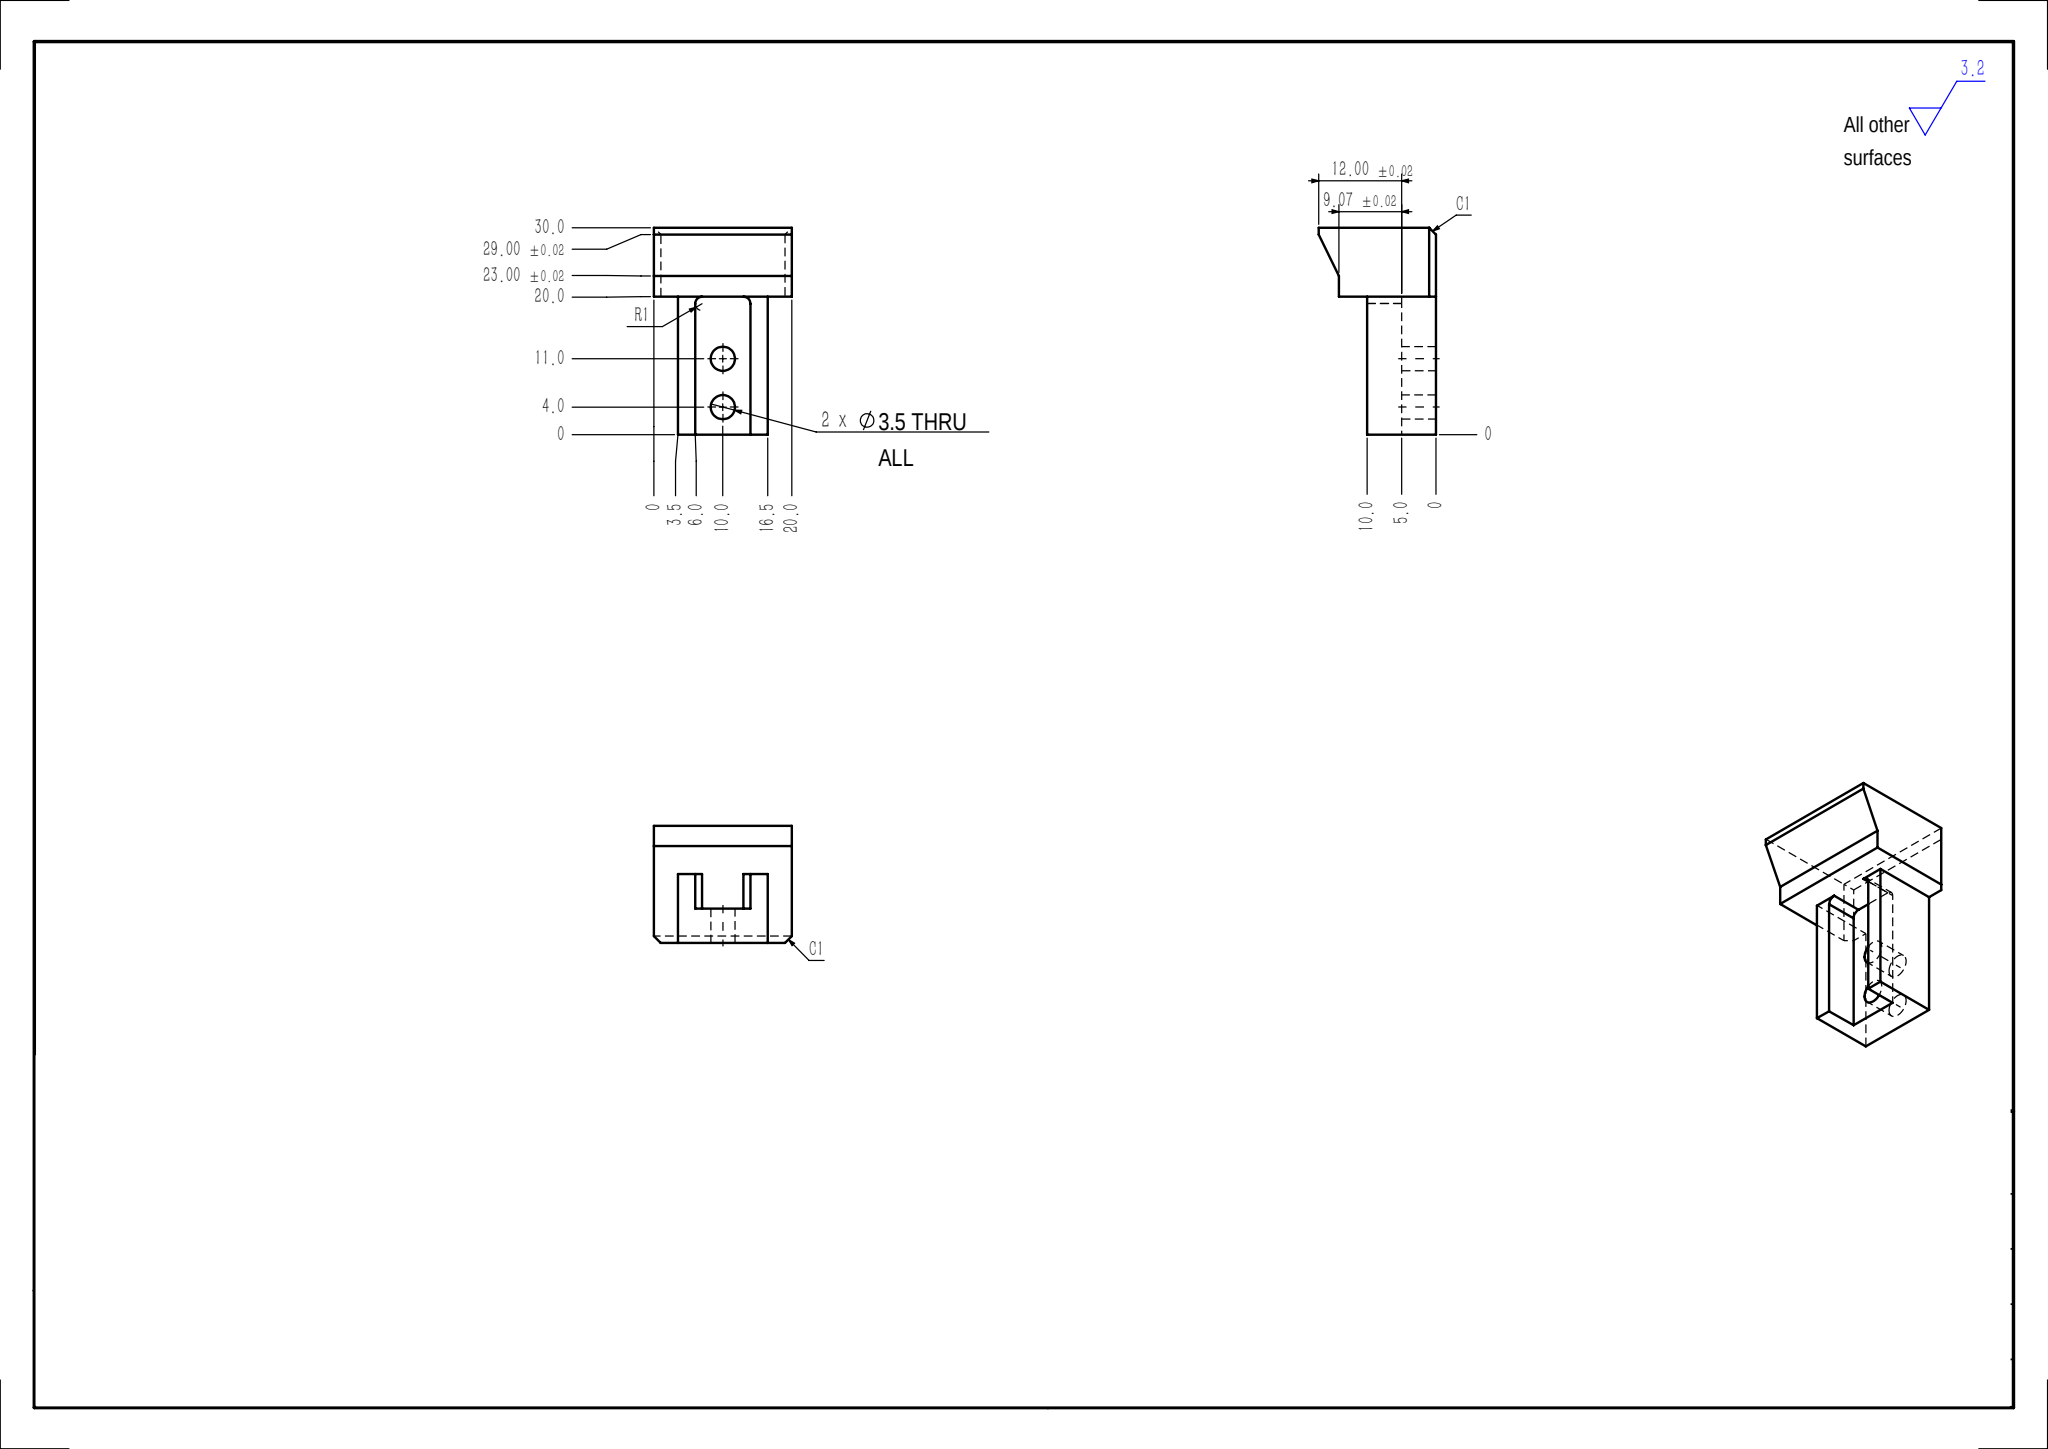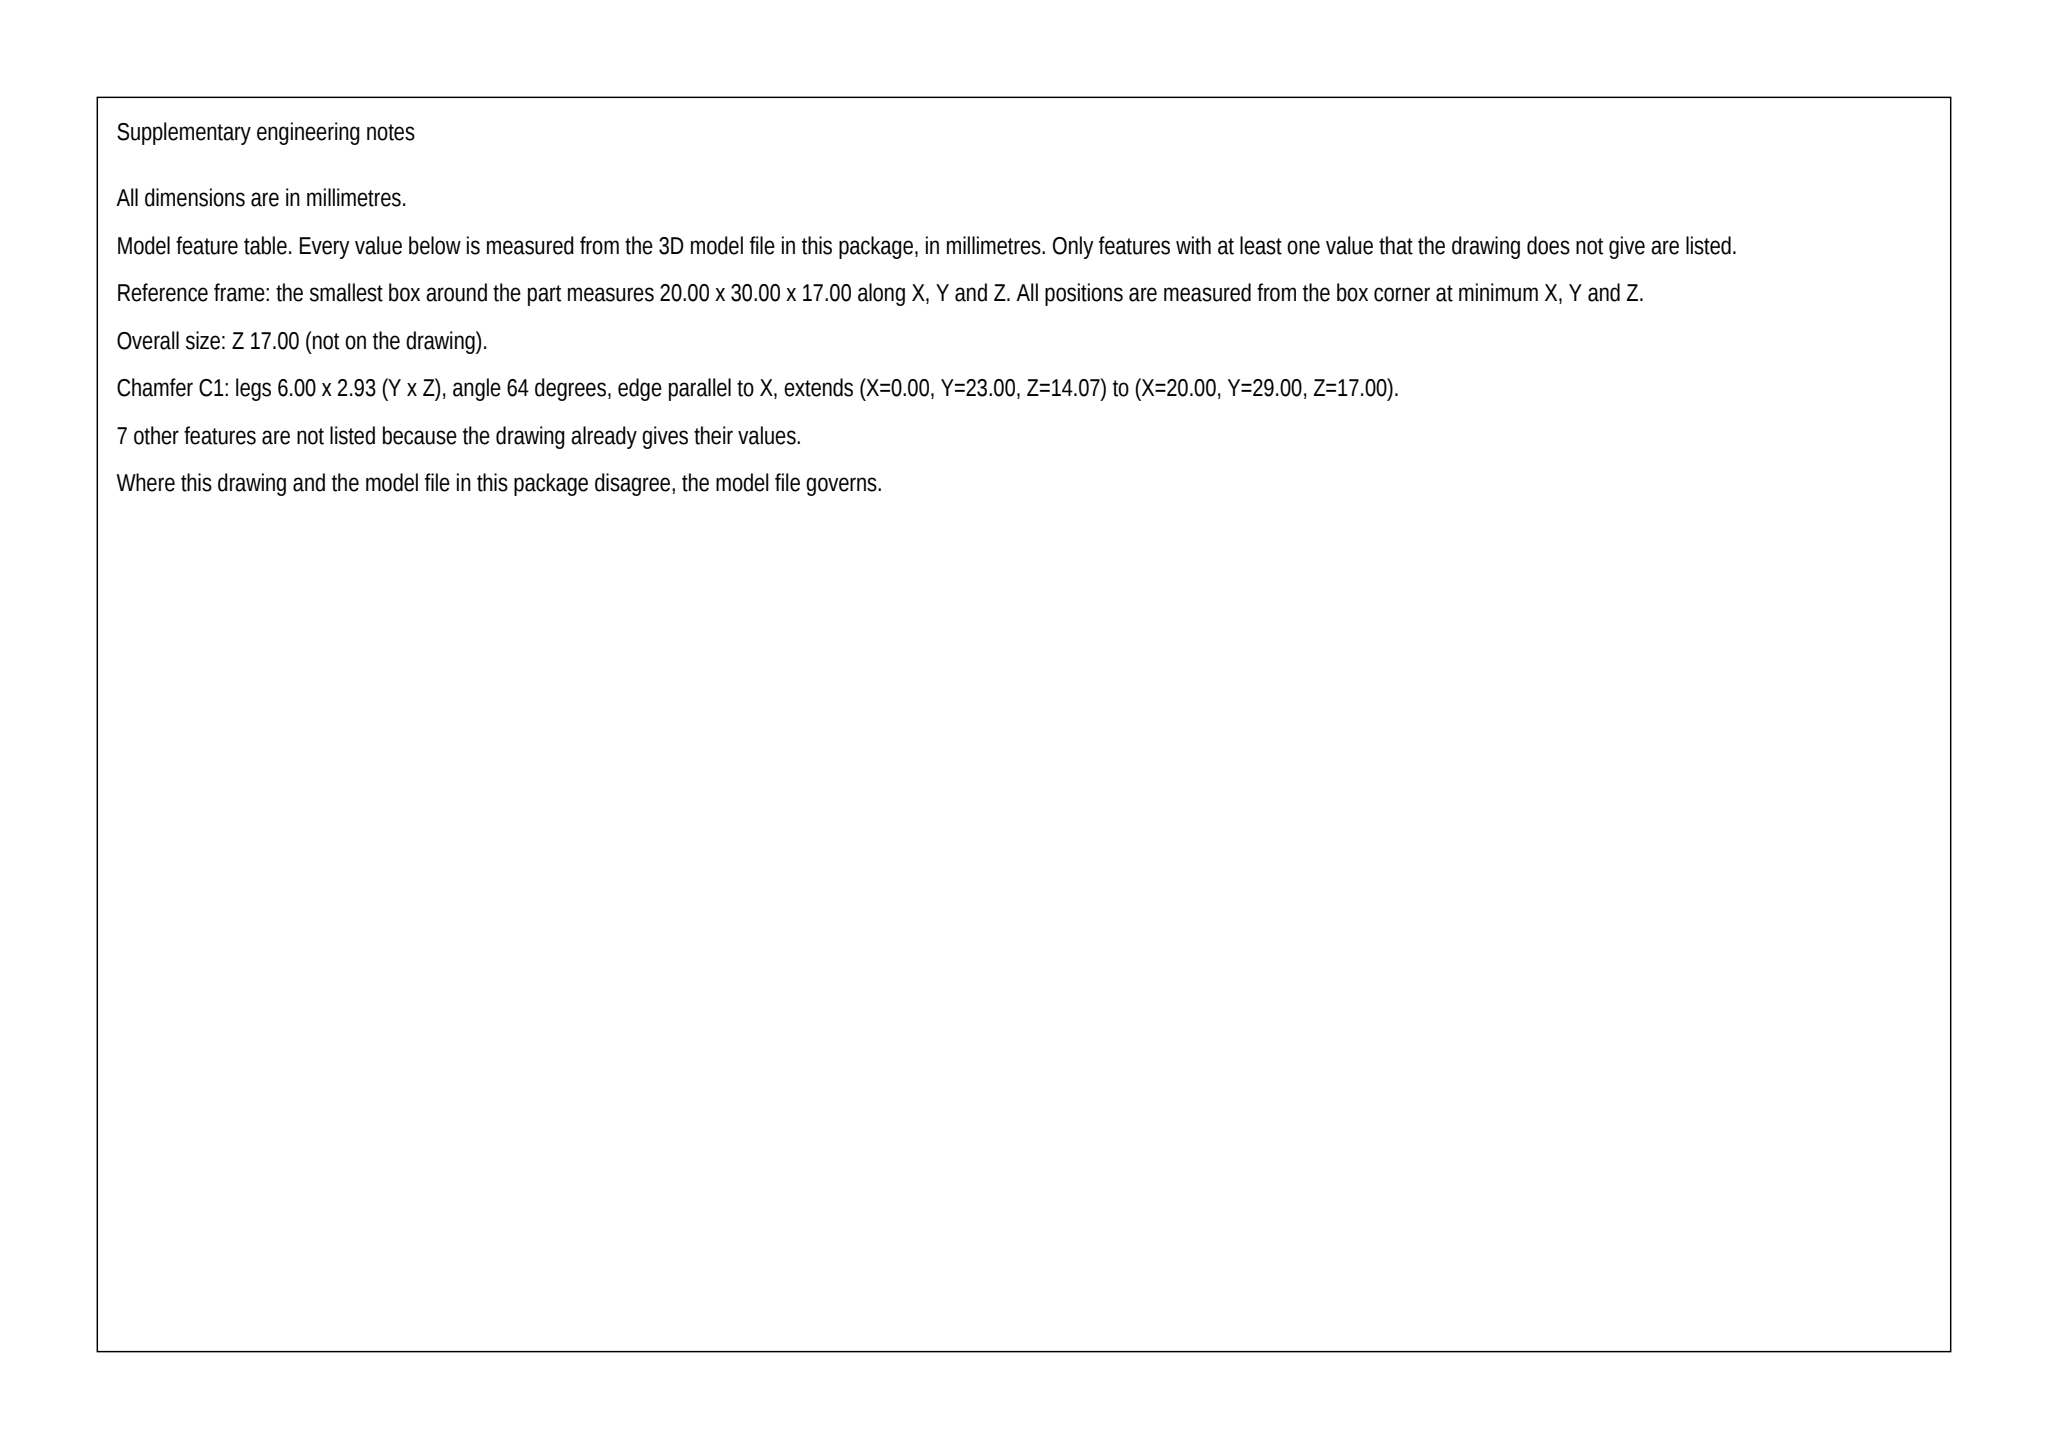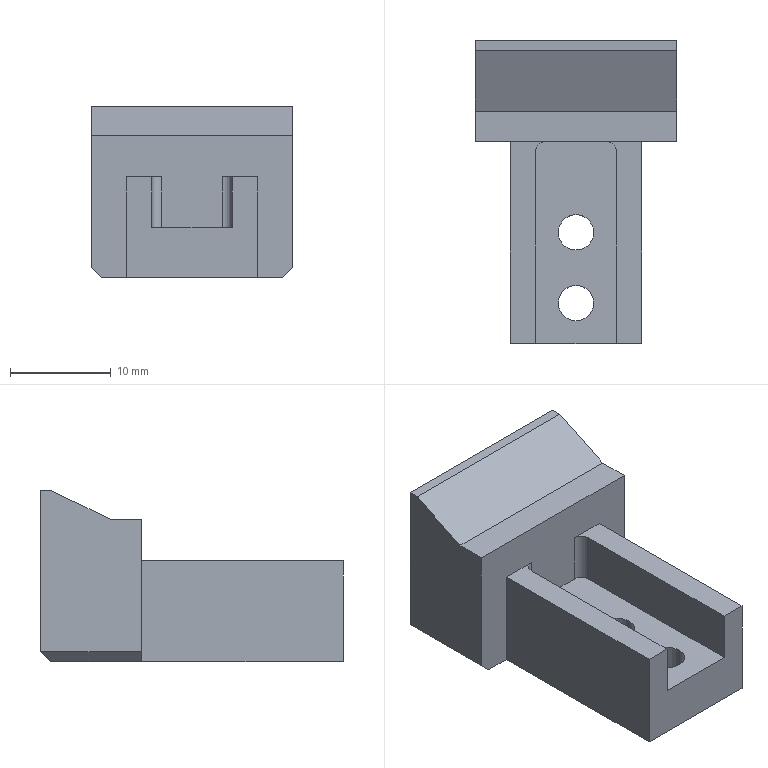Part | SolidWorks | mm | 1 solid | 25 faces | box 20 x 30 x 17 mm | volume 4735 mm3 | plane 19 | cylinder 6 | commonest cylinder face diameters 3.5 x4 2 x2
build123d program:
from build123d import *

# Parameters (mm, degrees)
SKETCH1_W                  = 20
SKETCH1_H                  = 30
BOSS_EXTRUDE1_DEPTH        = 5
SKETCH2_W                  = 8
SKETCH2_H                  = 40
CUT_EXTRUDE1_DEPTH         = 5
SKETCH3_W                  = 3.5
SKETCH3_H                  = 20
CUT_EXTRUDE2_DEPTH         = 21.616
SKETCH4_W                  = 20
SKETCH4_H                  = 10
BOSS_EXTRUDE2_DEPTH        = 8
F_3_5_3_5_DIAMETER_HOLE1_D = 3.5
CHAMFER1_SIZE              = 1
SKETCH8_W                  = 20
SKETCH8_H                  = 10
CUT_EXTRUDE4_DEPTH         = 1
FILLET3_R                  = 1
CUT_EXTRUDE5_DEPTH         = 28.731


with BuildPart() as part:
    # Sketch1 → Boss-Extrude1 (new, symmetric)
    with BuildSketch(Plane.XY):
        Rectangle(SKETCH1_W, SKETCH1_H)
    extrude(amount=BOSS_EXTRUDE1_DEPTH, both=True)

    # Sketch2 → Cut-Extrude1 (cut)
    with BuildSketch(Plane.XY.offset(5)):
        with Locations((0, -15)):
            Rectangle(SKETCH2_W, SKETCH2_H)
    extrude(amount=-CUT_EXTRUDE1_DEPTH, mode=Mode.SUBTRACT)

    # Sketch3 → Cut-Extrude2 (cut, through all)
    with BuildSketch(Plane.XY.offset(5)):
        with Locations((-8.25, -5)):
            Rectangle(SKETCH3_W, SKETCH3_H)
        with Locations((8.25, -5)):
            Rectangle(SKETCH3_W, SKETCH3_H)
    extrude(amount=-CUT_EXTRUDE2_DEPTH, mode=Mode.SUBTRACT)

    # Sketch4 → Boss-Extrude2 (add)
    with BuildSketch(Plane.XY.offset(5)):
        with Locations((0, 10)):
            Rectangle(SKETCH4_W, SKETCH4_H)
    extrude(amount=BOSS_EXTRUDE2_DEPTH)

    # 3.5 _3.5_ Diameter Hole1 (through all)
    with Locations(Plane(origin=(0, 0, -5), x_dir=(-1, 0, 0), z_dir=(0, 0, -1))):
        with Locations((0, -11), (0, -4)):
            Hole(F_3_5_3_5_DIAMETER_HOLE1_D / 2)

    # Chamfer1
    chamfer1_edges = [part.edges().sort_by_distance(p)[0] for p in [
        (10, 10, -5),
        (-10, 10, -5),
        (0, 15, -5),
    ]]
    chamfer(chamfer1_edges, length=CHAMFER1_SIZE)

    # Sketch8 → Cut-Extrude4 (cut)
    with BuildSketch(Plane.XY.offset(13)):
        with Locations((0, 10)):
            Rectangle(SKETCH8_W, SKETCH8_H)
    extrude(amount=-CUT_EXTRUDE4_DEPTH, mode=Mode.SUBTRACT)

    # Fillet3
    fillet3_edges = [part.edges().sort_by_distance(p)[0] for p in [
        (4, 5, 2.5),
        (-4, 5, 2.5),
    ]]
    fillet(fillet3_edges, radius=FILLET3_R)

    # Sketch9 → Cut-Extrude5 (cut, through all)
    with BuildSketch(Plane(origin=(10, 0, 0), x_dir=(0, 0, -1), z_dir=(1, 0, 0))):
        Polygon((-12, 14), (-9.074, 8), (-9.074, 5), (-12, 5), align=None)
    extrude(amount=-CUT_EXTRUDE5_DEPTH, mode=Mode.SUBTRACT)


solid = part.part
STEP:
#1=CARTESIAN_POINT('',(1.75,-11.,0.));
#2=VERTEX_POINT('',#1);
#3=CARTESIAN_POINT('',(-1.75,-11.,0.));
#4=VERTEX_POINT('',#3);
#5=CARTESIAN_POINT('',(-0.,-11.,0.));
#6=DIRECTION('',(0.,0.,-1.));
#7=DIRECTION('',(-1.,0.,0.));
#8=AXIS2_PLACEMENT_3D('',#5,#6,#7);
#9=CIRCLE('',#8,1.75);
#10=EDGE_CURVE('',#2,#4,#9,.T.);
#11=ORIENTED_EDGE('',*,*,#10,.F.);
#12=CARTESIAN_POINT('',(1.75,-11.,-5.));
#13=VERTEX_POINT('',#12);
#14=CARTESIAN_POINT('',(1.75,-11.,-5.));
#15=DIRECTION('',(0.,0.,-1.));
#16=VECTOR('',#15,1000.);
#17=LINE('',#14,#16);
#18=EDGE_CURVE('',#2,#13,#17,.T.);
#19=ORIENTED_EDGE('',*,*,#18,.T.);
#20=CARTESIAN_POINT('',(-1.75,-11.,-5.));
#21=VERTEX_POINT('',#20);
#22=CARTESIAN_POINT('',(-0.,-11.,-5.));
#23=DIRECTION('',(0.,0.,-1.));
#24=DIRECTION('',(-1.,0.,0.));
#25=AXIS2_PLACEMENT_3D('',#22,#23,#24);
#26=CIRCLE('',#25,1.75);
#27=EDGE_CURVE('',#13,#21,#26,.T.);
#28=ORIENTED_EDGE('',*,*,#27,.T.);
#29=CARTESIAN_POINT('',(-1.75,-11.,-5.));
#30=DIRECTION('',(0.,0.,-1.));
#31=VECTOR('',#30,1000.);
#32=LINE('',#29,#31);
#33=EDGE_CURVE('',#4,#21,#32,.T.);
#34=ORIENTED_EDGE('',*,*,#33,.F.);
#35=EDGE_LOOP('',(#11,#19,#28,#34));
#36=FACE_OUTER_BOUND('',#35,.T.);
#37=CARTESIAN_POINT('',(-0.,-11.,-5.));
#38=DIRECTION('',(0.,0.,-1.));
#39=DIRECTION('',(-1.,0.,0.));
#40=AXIS2_PLACEMENT_3D('',#37,#38,#39);
#41=CYLINDRICAL_SURFACE('',#40,1.75);
#42=ADVANCED_FACE('',(#36),#41,.F.);
#43=CARTESIAN_POINT('',(1.75,-4.,0.));
#44=VERTEX_POINT('',#43);
#45=CARTESIAN_POINT('',(-1.75,-4.,0.));
#46=VERTEX_POINT('',#45);
#47=CARTESIAN_POINT('',(0.,-4.,0.));
#48=DIRECTION('',(0.,0.,-1.));
#49=DIRECTION('',(-1.,0.,0.));
#50=AXIS2_PLACEMENT_3D('',#47,#48,#49);
#51=CIRCLE('',#50,1.75);
#52=EDGE_CURVE('',#44,#46,#51,.T.);
#53=ORIENTED_EDGE('',*,*,#52,.F.);
#54=CARTESIAN_POINT('',(1.75,-4.,-5.));
#55=VERTEX_POINT('',#54);
#56=CARTESIAN_POINT('',(1.75,-4.,-5.));
#57=DIRECTION('',(0.,0.,-1.));
#58=VECTOR('',#57,1000.);
#59=LINE('',#56,#58);
#60=EDGE_CURVE('',#44,#55,#59,.T.);
#61=ORIENTED_EDGE('',*,*,#60,.T.);
#62=CARTESIAN_POINT('',(-1.75,-4.,-5.));
#63=VERTEX_POINT('',#62);
#64=CARTESIAN_POINT('',(0.,-4.,-5.));
#65=DIRECTION('',(0.,0.,-1.));
#66=DIRECTION('',(-1.,0.,0.));
#67=AXIS2_PLACEMENT_3D('',#64,#65,#66);
#68=CIRCLE('',#67,1.75);
#69=EDGE_CURVE('',#55,#63,#68,.T.);
#70=ORIENTED_EDGE('',*,*,#69,.T.);
#71=CARTESIAN_POINT('',(-1.75,-4.,-5.));
#72=DIRECTION('',(0.,0.,-1.));
#73=VECTOR('',#72,1000.);
#74=LINE('',#71,#73);
#75=EDGE_CURVE('',#46,#63,#74,.T.);
#76=ORIENTED_EDGE('',*,*,#75,.F.);
#77=EDGE_LOOP('',(#53,#61,#70,#76));
#78=FACE_OUTER_BOUND('',#77,.T.);
#79=CARTESIAN_POINT('',(0.,-4.,-5.));
#80=DIRECTION('',(0.,0.,-1.));
#81=DIRECTION('',(-1.,0.,0.));
#82=AXIS2_PLACEMENT_3D('',#79,#80,#81);
#83=CYLINDRICAL_SURFACE('',#82,1.75);
#84=ADVANCED_FACE('',(#78),#83,.F.);
#85=CARTESIAN_POINT('',(10.,14.,12.));
#86=VERTEX_POINT('',#85);
#87=CARTESIAN_POINT('',(10.,15.,12.));
#88=VERTEX_POINT('',#87);
#89=CARTESIAN_POINT('',(10.,15.,12.));
#90=DIRECTION('',(0.,1.,0.));
#91=VECTOR('',#90,1000.);
#92=LINE('',#89,#91);
#93=EDGE_CURVE('',#86,#88,#92,.T.);
#94=ORIENTED_EDGE('',*,*,#93,.F.);
#95=CARTESIAN_POINT('',(10.,8.,9.074));
#96=VERTEX_POINT('',#95);
#97=CARTESIAN_POINT('',(10.,14.,12.));
#98=DIRECTION('',(0.,0.8988,0.4384));
#99=VECTOR('',#98,1000.);
#100=LINE('',#97,#99);
#101=EDGE_CURVE('',#96,#86,#100,.T.);
#102=ORIENTED_EDGE('',*,*,#101,.F.);
#103=CARTESIAN_POINT('',(10.,5.,9.074));
#104=VERTEX_POINT('',#103);
#105=CARTESIAN_POINT('',(10.,8.,9.074));
#106=DIRECTION('',(-0.,1.,0.));
#107=VECTOR('',#106,1000.);
#108=LINE('',#105,#107);
#109=EDGE_CURVE('',#104,#96,#108,.T.);
#110=ORIENTED_EDGE('',*,*,#109,.F.);
#111=CARTESIAN_POINT('',(10.,5.,-4.));
#112=VERTEX_POINT('',#111);
#113=CARTESIAN_POINT('',(10.,5.,-5.));
#114=DIRECTION('',(0.,0.,1.));
#115=VECTOR('',#114,1000.);
#116=LINE('',#113,#115);
#117=EDGE_CURVE('',#112,#104,#116,.T.);
#118=ORIENTED_EDGE('',*,*,#117,.F.);
#119=CARTESIAN_POINT('',(10.,15.,-4.));
#120=VERTEX_POINT('',#119);
#121=CARTESIAN_POINT('',(10.,15.,-4.));
#122=DIRECTION('',(-0.,1.,0.));
#123=VECTOR('',#122,1000.);
#124=LINE('',#121,#123);
#125=EDGE_CURVE('',#112,#120,#124,.T.);
#126=ORIENTED_EDGE('',*,*,#125,.T.);
#127=CARTESIAN_POINT('',(10.,15.,5.));
#128=DIRECTION('',(0.,0.,-1.));
#129=VECTOR('',#128,1000.);
#130=LINE('',#127,#129);
#131=EDGE_CURVE('',#88,#120,#130,.T.);
#132=ORIENTED_EDGE('',*,*,#131,.F.);
#133=EDGE_LOOP('',(#94,#102,#110,#118,#126,#132));
#134=FACE_OUTER_BOUND('',#133,.T.);
#135=CARTESIAN_POINT('',(10.,15.,5.));
#136=DIRECTION('',(-1.,-0.,0.));
#137=DIRECTION('',(0.,-1.,0.));
#138=AXIS2_PLACEMENT_3D('',#135,#136,#137);
#139=PLANE('',#138);
#140=ADVANCED_FACE('',(#134),#139,.F.);
#141=CARTESIAN_POINT('',(-10.,15.,12.));
#142=VERTEX_POINT('',#141);
#143=CARTESIAN_POINT('',(-10.,15.,12.));
#144=DIRECTION('',(-1.,0.,0.));
#145=VECTOR('',#144,1000.);
#146=LINE('',#143,#145);
#147=EDGE_CURVE('',#88,#142,#146,.T.);
#148=ORIENTED_EDGE('',*,*,#147,.F.);
#149=ORIENTED_EDGE('',*,*,#131,.T.);
#150=CARTESIAN_POINT('',(-10.,15.,-4.));
#151=VERTEX_POINT('',#150);
#152=CARTESIAN_POINT('',(-10.,15.,-4.));
#153=DIRECTION('',(-1.,0.,0.));
#154=VECTOR('',#153,1000.);
#155=LINE('',#152,#154);
#156=EDGE_CURVE('',#120,#151,#155,.T.);
#157=ORIENTED_EDGE('',*,*,#156,.T.);
#158=CARTESIAN_POINT('',(-10.,15.,5.));
#159=DIRECTION('',(0.,0.,-1.));
#160=VECTOR('',#159,1000.);
#161=LINE('',#158,#160);
#162=EDGE_CURVE('',#142,#151,#161,.T.);
#163=ORIENTED_EDGE('',*,*,#162,.F.);
#164=EDGE_LOOP('',(#148,#149,#157,#163));
#165=FACE_OUTER_BOUND('',#164,.T.);
#166=CARTESIAN_POINT('',(-10.,15.,5.));
#167=DIRECTION('',(0.,-1.,0.));
#168=DIRECTION('',(0.,0.,-1.));
#169=AXIS2_PLACEMENT_3D('',#166,#167,#168);
#170=PLANE('',#169);
#171=ADVANCED_FACE('',(#165),#170,.F.);
#172=CARTESIAN_POINT('',(-10.,5.,9.074));
#173=VERTEX_POINT('',#172);
#174=CARTESIAN_POINT('',(-10.,8.,9.074));
#175=VERTEX_POINT('',#174);
#176=CARTESIAN_POINT('',(-10.,8.,9.074));
#177=DIRECTION('',(-0.,1.,0.));
#178=VECTOR('',#177,1000.);
#179=LINE('',#176,#178);
#180=EDGE_CURVE('',#173,#175,#179,.T.);
#181=ORIENTED_EDGE('',*,*,#180,.T.);
#182=CARTESIAN_POINT('',(-10.,14.,12.));
#183=VERTEX_POINT('',#182);
#184=CARTESIAN_POINT('',(-10.,14.,12.));
#185=DIRECTION('',(0.,0.8988,0.4384));
#186=VECTOR('',#185,1000.);
#187=LINE('',#184,#186);
#188=EDGE_CURVE('',#175,#183,#187,.T.);
#189=ORIENTED_EDGE('',*,*,#188,.T.);
#190=CARTESIAN_POINT('',(-10.,15.,12.));
#191=DIRECTION('',(0.,-1.,0.));
#192=VECTOR('',#191,1000.);
#193=LINE('',#190,#192);
#194=EDGE_CURVE('',#142,#183,#193,.T.);
#195=ORIENTED_EDGE('',*,*,#194,.F.);
#196=ORIENTED_EDGE('',*,*,#162,.T.);
#197=CARTESIAN_POINT('',(-10.,5.,-4.));
#198=VERTEX_POINT('',#197);
#199=CARTESIAN_POINT('',(-10.,15.,-4.));
#200=DIRECTION('',(0.,-1.,0.));
#201=VECTOR('',#200,1000.);
#202=LINE('',#199,#201);
#203=EDGE_CURVE('',#151,#198,#202,.T.);
#204=ORIENTED_EDGE('',*,*,#203,.T.);
#205=CARTESIAN_POINT('',(-10.,5.,-5.));
#206=DIRECTION('',(0.,0.,1.));
#207=VECTOR('',#206,1000.);
#208=LINE('',#205,#207);
#209=EDGE_CURVE('',#198,#173,#208,.T.);
#210=ORIENTED_EDGE('',*,*,#209,.T.);
#211=EDGE_LOOP('',(#181,#189,#195,#196,#204,#210));
#212=FACE_OUTER_BOUND('',#211,.T.);
#213=CARTESIAN_POINT('',(-10.,15.,5.));
#214=DIRECTION('',(1.,0.,0.));
#215=DIRECTION('',(-0.,1.,0.));
#216=AXIS2_PLACEMENT_3D('',#213,#214,#215);
#217=PLANE('',#216);
#218=ADVANCED_FACE('',(#212),#217,.F.);
#219=ORIENTED_EDGE('',*,*,#117,.T.);
#220=CARTESIAN_POINT('',(-10.,5.,9.074));
#221=DIRECTION('',(1.,0.,0.));
#222=VECTOR('',#221,1000.);
#223=LINE('',#220,#222);
#224=EDGE_CURVE('',#173,#104,#223,.T.);
#225=ORIENTED_EDGE('',*,*,#224,.F.);
#226=ORIENTED_EDGE('',*,*,#209,.F.);
#227=CARTESIAN_POINT('',(-9.,5.,-5.));
#228=VERTEX_POINT('',#227);
#229=CARTESIAN_POINT('',(-10.,5.,-4.));
#230=DIRECTION('',(0.7071,0.,-0.7071));
#231=VECTOR('',#230,1000.);
#232=LINE('',#229,#231);
#233=EDGE_CURVE('',#198,#228,#232,.T.);
#234=ORIENTED_EDGE('',*,*,#233,.T.);
#235=CARTESIAN_POINT('',(-6.5,5.,-5.));
#236=VERTEX_POINT('',#235);
#237=CARTESIAN_POINT('',(-10.,5.,-5.));
#238=DIRECTION('',(-1.,0.,0.));
#239=VECTOR('',#238,1000.);
#240=LINE('',#237,#239);
#241=EDGE_CURVE('',#236,#228,#240,.T.);
#242=ORIENTED_EDGE('',*,*,#241,.F.);
#243=CARTESIAN_POINT('',(-6.5,5.,5.));
#244=VERTEX_POINT('',#243);
#245=CARTESIAN_POINT('',(-6.5,5.,-5.));
#246=DIRECTION('',(0.,0.,1.));
#247=VECTOR('',#246,1000.);
#248=LINE('',#245,#247);
#249=EDGE_CURVE('',#236,#244,#248,.T.);
#250=ORIENTED_EDGE('',*,*,#249,.T.);
#251=CARTESIAN_POINT('',(-3.,5.,5.));
#252=VERTEX_POINT('',#251);
#253=CARTESIAN_POINT('',(-10.,5.,5.));
#254=DIRECTION('',(1.,0.,0.));
#255=VECTOR('',#254,1000.);
#256=LINE('',#253,#255);
#257=EDGE_CURVE('',#244,#252,#256,.T.);
#258=ORIENTED_EDGE('',*,*,#257,.T.);
#259=CARTESIAN_POINT('',(-3.,5.,0.));
#260=VERTEX_POINT('',#259);
#261=CARTESIAN_POINT('',(-3.,5.,0.));
#262=DIRECTION('',(0.,0.,-1.));
#263=VECTOR('',#262,1000.);
#264=LINE('',#261,#263);
#265=EDGE_CURVE('',#252,#260,#264,.T.);
#266=ORIENTED_EDGE('',*,*,#265,.T.);
#267=CARTESIAN_POINT('',(3.,5.,0.));
#268=VERTEX_POINT('',#267);
#269=CARTESIAN_POINT('',(-4.,5.,0.));
#270=DIRECTION('',(-1.,-0.,0.));
#271=VECTOR('',#270,1000.);
#272=LINE('',#269,#271);
#273=EDGE_CURVE('',#268,#260,#272,.T.);
#274=ORIENTED_EDGE('',*,*,#273,.F.);
#275=CARTESIAN_POINT('',(3.,5.,5.));
#276=VERTEX_POINT('',#275);
#277=CARTESIAN_POINT('',(3.,5.,5.));
#278=DIRECTION('',(0.,0.,1.));
#279=VECTOR('',#278,1000.);
#280=LINE('',#277,#279);
#281=EDGE_CURVE('',#268,#276,#280,.T.);
#282=ORIENTED_EDGE('',*,*,#281,.T.);
#283=CARTESIAN_POINT('',(6.5,5.,5.));
#284=VERTEX_POINT('',#283);
#285=CARTESIAN_POINT('',(-10.,5.,5.));
#286=DIRECTION('',(1.,0.,0.));
#287=VECTOR('',#286,1000.);
#288=LINE('',#285,#287);
#289=EDGE_CURVE('',#276,#284,#288,.T.);
#290=ORIENTED_EDGE('',*,*,#289,.T.);
#291=CARTESIAN_POINT('',(6.5,5.,-5.));
#292=VERTEX_POINT('',#291);
#293=CARTESIAN_POINT('',(6.5,5.,-5.));
#294=DIRECTION('',(0.,0.,1.));
#295=VECTOR('',#294,1000.);
#296=LINE('',#293,#295);
#297=EDGE_CURVE('',#292,#284,#296,.T.);
#298=ORIENTED_EDGE('',*,*,#297,.F.);
#299=CARTESIAN_POINT('',(9.,5.,-5.));
#300=VERTEX_POINT('',#299);
#301=CARTESIAN_POINT('',(10.,5.,-5.));
#302=DIRECTION('',(-1.,0.,0.));
#303=VECTOR('',#302,1000.);
#304=LINE('',#301,#303);
#305=EDGE_CURVE('',#300,#292,#304,.T.);
#306=ORIENTED_EDGE('',*,*,#305,.F.);
#307=CARTESIAN_POINT('',(10.,5.,-4.));
#308=DIRECTION('',(0.7071,0.,0.7071));
#309=VECTOR('',#308,1000.);
#310=LINE('',#307,#309);
#311=EDGE_CURVE('',#300,#112,#310,.T.);
#312=ORIENTED_EDGE('',*,*,#311,.T.);
#313=EDGE_LOOP('',(#219,#225,#226,#234,#242,#250,#258,#266,#274,#282,#290,#298,#306,#312));
#314=FACE_OUTER_BOUND('',#313,.T.);
#315=CARTESIAN_POINT('',(-4.,5.,0.));
#316=DIRECTION('',(-0.,1.,0.));
#317=DIRECTION('',(-1.,-0.,0.));
#318=AXIS2_PLACEMENT_3D('',#315,#316,#317);
#319=PLANE('',#318);
#320=ADVANCED_FACE('',(#314),#319,.F.);
#321=ORIENTED_EDGE('',*,*,#257,.F.);
#322=CARTESIAN_POINT('',(-6.5,-15.,5.));
#323=VERTEX_POINT('',#322);
#324=CARTESIAN_POINT('',(-6.5,-15.,5.));
#325=DIRECTION('',(0.,1.,0.));
#326=VECTOR('',#325,1000.);
#327=LINE('',#324,#326);
#328=EDGE_CURVE('',#323,#244,#327,.T.);
#329=ORIENTED_EDGE('',*,*,#328,.F.);
#330=CARTESIAN_POINT('',(-4.,-15.,5.));
#331=VERTEX_POINT('',#330);
#332=CARTESIAN_POINT('',(-10.,-15.,5.));
#333=DIRECTION('',(1.,0.,0.));
#334=VECTOR('',#333,1000.);
#335=LINE('',#332,#334);
#336=EDGE_CURVE('',#323,#331,#335,.T.);
#337=ORIENTED_EDGE('',*,*,#336,.T.);
#338=CARTESIAN_POINT('',(-4.,4.,5.));
#339=VERTEX_POINT('',#338);
#340=CARTESIAN_POINT('',(-4.,-35.,5.));
#341=DIRECTION('',(0.,-1.,0.));
#342=VECTOR('',#341,1000.);
#343=LINE('',#340,#342);
#344=EDGE_CURVE('',#339,#331,#343,.T.);
#345=ORIENTED_EDGE('',*,*,#344,.F.);
#346=CARTESIAN_POINT('',(-3.,4.,5.));
#347=DIRECTION('',(0.,0.,-1.));
#348=DIRECTION('',(1.,0.,0.));
#349=AXIS2_PLACEMENT_3D('',#346,#347,#348);
#350=CIRCLE('',#349,1.);
#351=EDGE_CURVE('',#339,#252,#350,.T.);
#352=ORIENTED_EDGE('',*,*,#351,.T.);
#353=EDGE_LOOP('',(#321,#329,#337,#345,#352));
#354=FACE_OUTER_BOUND('',#353,.T.);
#355=CARTESIAN_POINT('',(0.,0.,5.));
#356=DIRECTION('',(0.,0.,1.));
#357=DIRECTION('',(1.,0.,0.));
#358=AXIS2_PLACEMENT_3D('',#355,#356,#357);
#359=PLANE('',#358);
#360=ADVANCED_FACE('',(#354),#359,.T.);
#361=ORIENTED_EDGE('',*,*,#336,.F.);
#362=CARTESIAN_POINT('',(-6.5,-15.,-5.));
#363=VERTEX_POINT('',#362);
#364=CARTESIAN_POINT('',(-6.5,-15.,-5.));
#365=DIRECTION('',(0.,0.,1.));
#366=VECTOR('',#365,1000.);
#367=LINE('',#364,#366);
#368=EDGE_CURVE('',#363,#323,#367,.T.);
#369=ORIENTED_EDGE('',*,*,#368,.F.);
#370=CARTESIAN_POINT('',(6.5,-15.,-5.));
#371=VERTEX_POINT('',#370);
#372=CARTESIAN_POINT('',(-10.,-15.,-5.));
#373=DIRECTION('',(1.,0.,0.));
#374=VECTOR('',#373,1000.);
#375=LINE('',#372,#374);
#376=EDGE_CURVE('',#363,#371,#375,.T.);
#377=ORIENTED_EDGE('',*,*,#376,.T.);
#378=CARTESIAN_POINT('',(6.5,-15.,5.));
#379=VERTEX_POINT('',#378);
#380=CARTESIAN_POINT('',(6.5,-15.,-5.));
#381=DIRECTION('',(0.,0.,1.));
#382=VECTOR('',#381,1000.);
#383=LINE('',#380,#382);
#384=EDGE_CURVE('',#371,#379,#383,.T.);
#385=ORIENTED_EDGE('',*,*,#384,.T.);
#386=CARTESIAN_POINT('',(4.,-15.,5.));
#387=VERTEX_POINT('',#386);
#388=CARTESIAN_POINT('',(-10.,-15.,5.));
#389=DIRECTION('',(1.,0.,0.));
#390=VECTOR('',#389,1000.);
#391=LINE('',#388,#390);
#392=EDGE_CURVE('',#387,#379,#391,.T.);
#393=ORIENTED_EDGE('',*,*,#392,.F.);
#394=CARTESIAN_POINT('',(4.,-15.,0.));
#395=VERTEX_POINT('',#394);
#396=CARTESIAN_POINT('',(4.,-15.,5.));
#397=DIRECTION('',(0.,0.,-1.));
#398=VECTOR('',#397,1000.);
#399=LINE('',#396,#398);
#400=EDGE_CURVE('',#387,#395,#399,.T.);
#401=ORIENTED_EDGE('',*,*,#400,.T.);
#402=CARTESIAN_POINT('',(-4.,-15.,0.));
#403=VERTEX_POINT('',#402);
#404=CARTESIAN_POINT('',(-10.,-15.,0.));
#405=DIRECTION('',(-1.,0.,0.));
#406=VECTOR('',#405,1000.);
#407=LINE('',#404,#406);
#408=EDGE_CURVE('',#395,#403,#407,.T.);
#409=ORIENTED_EDGE('',*,*,#408,.T.);
#410=CARTESIAN_POINT('',(-4.,-15.,5.));
#411=DIRECTION('',(0.,0.,1.));
#412=VECTOR('',#411,1000.);
#413=LINE('',#410,#412);
#414=EDGE_CURVE('',#403,#331,#413,.T.);
#415=ORIENTED_EDGE('',*,*,#414,.T.);
#416=EDGE_LOOP('',(#361,#369,#377,#385,#393,#401,#409,#415));
#417=FACE_OUTER_BOUND('',#416,.T.);
#418=CARTESIAN_POINT('',(-10.,-15.,5.));
#419=DIRECTION('',(0.,1.,0.));
#420=DIRECTION('',(0.,0.,1.));
#421=AXIS2_PLACEMENT_3D('',#418,#419,#420);
#422=PLANE('',#421);
#423=ADVANCED_FACE('',(#417),#422,.F.);
#424=ORIENTED_EDGE('',*,*,#289,.F.);
#425=CARTESIAN_POINT('',(4.,4.,5.));
#426=VERTEX_POINT('',#425);
#427=CARTESIAN_POINT('',(3.,4.,5.));
#428=DIRECTION('',(0.,0.,-1.));
#429=DIRECTION('',(1.,0.,0.));
#430=AXIS2_PLACEMENT_3D('',#427,#428,#429);
#431=CIRCLE('',#430,1.);
#432=EDGE_CURVE('',#276,#426,#431,.T.);
#433=ORIENTED_EDGE('',*,*,#432,.T.);
#434=CARTESIAN_POINT('',(4.,0.,5.));
#435=DIRECTION('',(0.,1.,0.));
#436=VECTOR('',#435,1000.);
#437=LINE('',#434,#436);
#438=EDGE_CURVE('',#387,#426,#437,.T.);
#439=ORIENTED_EDGE('',*,*,#438,.F.);
#440=ORIENTED_EDGE('',*,*,#392,.T.);
#441=CARTESIAN_POINT('',(6.5,-15.,5.));
#442=DIRECTION('',(0.,-1.,0.));
#443=VECTOR('',#442,1000.);
#444=LINE('',#441,#443);
#445=EDGE_CURVE('',#284,#379,#444,.T.);
#446=ORIENTED_EDGE('',*,*,#445,.F.);
#447=EDGE_LOOP('',(#424,#433,#439,#440,#446));
#448=FACE_OUTER_BOUND('',#447,.T.);
#449=CARTESIAN_POINT('',(0.,0.,5.));
#450=DIRECTION('',(0.,0.,1.));
#451=DIRECTION('',(1.,0.,0.));
#452=AXIS2_PLACEMENT_3D('',#449,#450,#451);
#453=PLANE('',#452);
#454=ADVANCED_FACE('',(#448),#453,.T.);
#455=CARTESIAN_POINT('',(-0.,-11.,-5.));
#456=DIRECTION('',(0.,0.,-1.));
#457=DIRECTION('',(-1.,0.,0.));
#458=AXIS2_PLACEMENT_3D('',#455,#456,#457);
#459=CIRCLE('',#458,1.75);
#460=EDGE_CURVE('',#21,#13,#459,.T.);
#461=ORIENTED_EDGE('',*,*,#460,.F.);
#462=ORIENTED_EDGE('',*,*,#27,.F.);
#463=EDGE_LOOP('',(#461,#462));
#464=FACE_BOUND('',#463,.T.);
#465=CARTESIAN_POINT('',(0.,-4.,-5.));
#466=DIRECTION('',(0.,0.,-1.));
#467=DIRECTION('',(-1.,0.,0.));
#468=AXIS2_PLACEMENT_3D('',#465,#466,#467);
#469=CIRCLE('',#468,1.75);
#470=EDGE_CURVE('',#63,#55,#469,.T.);
#471=ORIENTED_EDGE('',*,*,#470,.F.);
#472=ORIENTED_EDGE('',*,*,#69,.F.);
#473=EDGE_LOOP('',(#471,#472));
#474=FACE_BOUND('',#473,.T.);
#475=CARTESIAN_POINT('',(-9.,14.,-5.));
#476=VERTEX_POINT('',#475);
#477=CARTESIAN_POINT('',(9.,14.,-5.));
#478=VERTEX_POINT('',#477);
#479=CARTESIAN_POINT('',(0.,14.,-5.));
#480=DIRECTION('',(1.,0.,0.));
#481=VECTOR('',#480,1000.);
#482=LINE('',#479,#481);
#483=EDGE_CURVE('',#476,#478,#482,.T.);
#484=ORIENTED_EDGE('',*,*,#483,.T.);
#485=CARTESIAN_POINT('',(9.,0.,-5.));
#486=DIRECTION('',(0.,-1.,0.));
#487=VECTOR('',#486,1000.);
#488=LINE('',#485,#487);
#489=EDGE_CURVE('',#478,#300,#488,.T.);
#490=ORIENTED_EDGE('',*,*,#489,.T.);
#491=ORIENTED_EDGE('',*,*,#305,.T.);
#492=CARTESIAN_POINT('',(6.5,-15.,-5.));
#493=DIRECTION('',(0.,-1.,0.));
#494=VECTOR('',#493,1000.);
#495=LINE('',#492,#494);
#496=EDGE_CURVE('',#292,#371,#495,.T.);
#497=ORIENTED_EDGE('',*,*,#496,.T.);
#498=ORIENTED_EDGE('',*,*,#376,.F.);
#499=CARTESIAN_POINT('',(-6.5,-15.,-5.));
#500=DIRECTION('',(0.,1.,0.));
#501=VECTOR('',#500,1000.);
#502=LINE('',#499,#501);
#503=EDGE_CURVE('',#363,#236,#502,.T.);
#504=ORIENTED_EDGE('',*,*,#503,.T.);
#505=ORIENTED_EDGE('',*,*,#241,.T.);
#506=CARTESIAN_POINT('',(-9.,-0.,-5.));
#507=DIRECTION('',(-0.,1.,0.));
#508=VECTOR('',#507,1000.);
#509=LINE('',#506,#508);
#510=EDGE_CURVE('',#228,#476,#509,.T.);
#511=ORIENTED_EDGE('',*,*,#510,.T.);
#512=EDGE_LOOP('',(#484,#490,#491,#497,#498,#504,#505,#511));
#513=FACE_OUTER_BOUND('',#512,.T.);
#514=CARTESIAN_POINT('',(0.,0.,-5.));
#515=DIRECTION('',(0.,0.,1.));
#516=DIRECTION('',(1.,0.,0.));
#517=AXIS2_PLACEMENT_3D('',#514,#515,#516);
#518=PLANE('',#517);
#519=ADVANCED_FACE('',(#464,#474,#513),#518,.F.);
#520=CARTESIAN_POINT('',(-0.,-11.,0.));
#521=DIRECTION('',(0.,0.,-1.));
#522=DIRECTION('',(-1.,0.,0.));
#523=AXIS2_PLACEMENT_3D('',#520,#521,#522);
#524=CIRCLE('',#523,1.75);
#525=EDGE_CURVE('',#4,#2,#524,.T.);
#526=ORIENTED_EDGE('',*,*,#525,.T.);
#527=ORIENTED_EDGE('',*,*,#10,.T.);
#528=EDGE_LOOP('',(#526,#527));
#529=FACE_BOUND('',#528,.T.);
#530=CARTESIAN_POINT('',(0.,-4.,0.));
#531=DIRECTION('',(0.,0.,-1.));
#532=DIRECTION('',(-1.,0.,0.));
#533=AXIS2_PLACEMENT_3D('',#530,#531,#532);
#534=CIRCLE('',#533,1.75);
#535=EDGE_CURVE('',#46,#44,#534,.T.);
#536=ORIENTED_EDGE('',*,*,#535,.T.);
#537=ORIENTED_EDGE('',*,*,#52,.T.);
#538=EDGE_LOOP('',(#536,#537));
#539=FACE_BOUND('',#538,.T.);
#540=CARTESIAN_POINT('',(4.,4.,0.));
#541=VERTEX_POINT('',#540);
#542=CARTESIAN_POINT('',(4.,-35.,0.));
#543=DIRECTION('',(0.,1.,0.));
#544=VECTOR('',#543,1000.);
#545=LINE('',#542,#544);
#546=EDGE_CURVE('',#395,#541,#545,.T.);
#547=ORIENTED_EDGE('',*,*,#546,.T.);
#548=CARTESIAN_POINT('',(3.,4.,0.));
#549=DIRECTION('',(0.,0.,1.));
#550=DIRECTION('',(-1.,0.,0.));
#551=AXIS2_PLACEMENT_3D('',#548,#549,#550);
#552=CIRCLE('',#551,1.);
#553=EDGE_CURVE('',#541,#268,#552,.T.);
#554=ORIENTED_EDGE('',*,*,#553,.T.);
#555=ORIENTED_EDGE('',*,*,#273,.T.);
#556=CARTESIAN_POINT('',(-4.,4.,0.));
#557=VERTEX_POINT('',#556);
#558=CARTESIAN_POINT('',(-3.,4.,0.));
#559=DIRECTION('',(0.,0.,1.));
#560=DIRECTION('',(-1.,0.,0.));
#561=AXIS2_PLACEMENT_3D('',#558,#559,#560);
#562=CIRCLE('',#561,1.);
#563=EDGE_CURVE('',#260,#557,#562,.T.);
#564=ORIENTED_EDGE('',*,*,#563,.T.);
#565=CARTESIAN_POINT('',(-4.,-35.,0.));
#566=DIRECTION('',(0.,-1.,0.));
#567=VECTOR('',#566,1000.);
#568=LINE('',#565,#567);
#569=EDGE_CURVE('',#557,#403,#568,.T.);
#570=ORIENTED_EDGE('',*,*,#569,.T.);
#571=ORIENTED_EDGE('',*,*,#408,.F.);
#572=EDGE_LOOP('',(#547,#554,#555,#564,#570,#571));
#573=FACE_OUTER_BOUND('',#572,.T.);
#574=CARTESIAN_POINT('',(0.,0.,0.));
#575=DIRECTION('',(0.,0.,-1.));
#576=DIRECTION('',(-1.,0.,0.));
#577=AXIS2_PLACEMENT_3D('',#574,#575,#576);
#578=PLANE('',#577);
#579=ADVANCED_FACE('',(#529,#539,#573),#578,.F.);
#580=ORIENTED_EDGE('',*,*,#438,.T.);
#581=CARTESIAN_POINT('',(4.,4.,0.));
#582=DIRECTION('',(0.,0.,-1.));
#583=VECTOR('',#582,1000.);
#584=LINE('',#581,#583);
#585=EDGE_CURVE('',#426,#541,#584,.T.);
#586=ORIENTED_EDGE('',*,*,#585,.T.);
#587=ORIENTED_EDGE('',*,*,#546,.F.);
#588=ORIENTED_EDGE('',*,*,#400,.F.);
#589=EDGE_LOOP('',(#580,#586,#587,#588));
#590=FACE_OUTER_BOUND('',#589,.T.);
#591=CARTESIAN_POINT('',(4.,-35.,0.));
#592=DIRECTION('',(1.,0.,0.));
#593=DIRECTION('',(0.,0.,-1.));
#594=AXIS2_PLACEMENT_3D('',#591,#592,#593);
#595=PLANE('',#594);
#596=ADVANCED_FACE('',(#590),#595,.F.);
#597=ORIENTED_EDGE('',*,*,#569,.F.);
#598=CARTESIAN_POINT('',(-4.,4.,5.));
#599=DIRECTION('',(0.,0.,1.));
#600=VECTOR('',#599,1000.);
#601=LINE('',#598,#600);
#602=EDGE_CURVE('',#557,#339,#601,.T.);
#603=ORIENTED_EDGE('',*,*,#602,.T.);
#604=ORIENTED_EDGE('',*,*,#344,.T.);
#605=ORIENTED_EDGE('',*,*,#414,.F.);
#606=EDGE_LOOP('',(#597,#603,#604,#605));
#607=FACE_OUTER_BOUND('',#606,.T.);
#608=CARTESIAN_POINT('',(-4.,-35.,0.));
#609=DIRECTION('',(-1.,0.,0.));
#610=DIRECTION('',(0.,0.,1.));
#611=AXIS2_PLACEMENT_3D('',#608,#609,#610);
#612=PLANE('',#611);
#613=ADVANCED_FACE('',(#607),#612,.F.);
#614=ORIENTED_EDGE('',*,*,#445,.T.);
#615=ORIENTED_EDGE('',*,*,#384,.F.);
#616=ORIENTED_EDGE('',*,*,#496,.F.);
#617=ORIENTED_EDGE('',*,*,#297,.T.);
#618=EDGE_LOOP('',(#614,#615,#616,#617));
#619=FACE_OUTER_BOUND('',#618,.T.);
#620=CARTESIAN_POINT('',(6.5,-15.,-5.));
#621=DIRECTION('',(-1.,0.,0.));
#622=DIRECTION('',(0.,0.,1.));
#623=AXIS2_PLACEMENT_3D('',#620,#621,#622);
#624=PLANE('',#623);
#625=ADVANCED_FACE('',(#619),#624,.F.);
#626=ORIENTED_EDGE('',*,*,#328,.T.);
#627=ORIENTED_EDGE('',*,*,#249,.F.);
#628=ORIENTED_EDGE('',*,*,#503,.F.);
#629=ORIENTED_EDGE('',*,*,#368,.T.);
#630=EDGE_LOOP('',(#626,#627,#628,#629));
#631=FACE_OUTER_BOUND('',#630,.T.);
#632=CARTESIAN_POINT('',(-6.5,-15.,-5.));
#633=DIRECTION('',(1.,0.,0.));
#634=DIRECTION('',(0.,0.,-1.));
#635=AXIS2_PLACEMENT_3D('',#632,#633,#634);
#636=PLANE('',#635);
#637=ADVANCED_FACE('',(#631),#636,.F.);
#638=ORIENTED_EDGE('',*,*,#60,.F.);
#639=ORIENTED_EDGE('',*,*,#535,.F.);
#640=ORIENTED_EDGE('',*,*,#75,.T.);
#641=ORIENTED_EDGE('',*,*,#470,.T.);
#642=EDGE_LOOP('',(#638,#639,#640,#641));
#643=FACE_OUTER_BOUND('',#642,.T.);
#644=CARTESIAN_POINT('',(0.,-4.,-5.));
#645=DIRECTION('',(0.,0.,-1.));
#646=DIRECTION('',(-1.,0.,0.));
#647=AXIS2_PLACEMENT_3D('',#644,#645,#646);
#648=CYLINDRICAL_SURFACE('',#647,1.75);
#649=ADVANCED_FACE('',(#643),#648,.F.);
#650=ORIENTED_EDGE('',*,*,#18,.F.);
#651=ORIENTED_EDGE('',*,*,#525,.F.);
#652=ORIENTED_EDGE('',*,*,#33,.T.);
#653=ORIENTED_EDGE('',*,*,#460,.T.);
#654=EDGE_LOOP('',(#650,#651,#652,#653));
#655=FACE_OUTER_BOUND('',#654,.T.);
#656=CARTESIAN_POINT('',(-0.,-11.,-5.));
#657=DIRECTION('',(0.,0.,-1.));
#658=DIRECTION('',(-1.,0.,0.));
#659=AXIS2_PLACEMENT_3D('',#656,#657,#658);
#660=CYLINDRICAL_SURFACE('',#659,1.75);
#661=ADVANCED_FACE('',(#655),#660,.F.);
#662=ORIENTED_EDGE('',*,*,#233,.F.);
#663=ORIENTED_EDGE('',*,*,#203,.F.);
#664=CARTESIAN_POINT('',(-10.,15.,-4.));
#665=DIRECTION('',(-0.5774,0.5774,0.5774));
#666=VECTOR('',#665,1000.);
#667=LINE('',#664,#666);
#668=EDGE_CURVE('',#476,#151,#667,.T.);
#669=ORIENTED_EDGE('',*,*,#668,.F.);
#670=ORIENTED_EDGE('',*,*,#510,.F.);
#671=EDGE_LOOP('',(#662,#663,#669,#670));
#672=FACE_OUTER_BOUND('',#671,.T.);
#673=CARTESIAN_POINT('',(-10.,15.,-4.));
#674=DIRECTION('',(0.7071,0.,0.7071));
#675=DIRECTION('',(0.,-1.,0.));
#676=AXIS2_PLACEMENT_3D('',#673,#674,#675);
#677=PLANE('',#676);
#678=ADVANCED_FACE('',(#672),#677,.F.);
#679=ORIENTED_EDGE('',*,*,#668,.T.);
#680=ORIENTED_EDGE('',*,*,#156,.F.);
#681=CARTESIAN_POINT('',(3.333,8.333,-10.667));
#682=DIRECTION('',(0.5774,0.5774,0.5774));
#683=VECTOR('',#682,1000.);
#684=LINE('',#681,#683);
#685=EDGE_CURVE('',#478,#120,#684,.T.);
#686=ORIENTED_EDGE('',*,*,#685,.F.);
#687=ORIENTED_EDGE('',*,*,#483,.F.);
#688=EDGE_LOOP('',(#679,#680,#686,#687));
#689=FACE_OUTER_BOUND('',#688,.T.);
#690=CARTESIAN_POINT('',(-10.,15.,-4.));
#691=DIRECTION('',(0.,-0.7071,0.7071));
#692=DIRECTION('',(-1.,0.,0.));
#693=AXIS2_PLACEMENT_3D('',#690,#691,#692);
#694=PLANE('',#693);
#695=ADVANCED_FACE('',(#689),#694,.F.);
#696=ORIENTED_EDGE('',*,*,#311,.F.);
#697=ORIENTED_EDGE('',*,*,#489,.F.);
#698=ORIENTED_EDGE('',*,*,#685,.T.);
#699=ORIENTED_EDGE('',*,*,#125,.F.);
#700=EDGE_LOOP('',(#696,#697,#698,#699));
#701=FACE_OUTER_BOUND('',#700,.T.);
#702=CARTESIAN_POINT('',(10.,15.,-4.));
#703=DIRECTION('',(-0.7071,-0.,0.7071));
#704=DIRECTION('',(-0.,1.,0.));
#705=AXIS2_PLACEMENT_3D('',#702,#703,#704);
#706=PLANE('',#705);
#707=ADVANCED_FACE('',(#701),#706,.F.);
#708=CARTESIAN_POINT('',(-10.,14.,12.));
#709=DIRECTION('',(1.,0.,0.));
#710=VECTOR('',#709,1000.);
#711=LINE('',#708,#710);
#712=EDGE_CURVE('',#183,#86,#711,.T.);
#713=ORIENTED_EDGE('',*,*,#712,.T.);
#714=ORIENTED_EDGE('',*,*,#93,.T.);
#715=ORIENTED_EDGE('',*,*,#147,.T.);
#716=ORIENTED_EDGE('',*,*,#194,.T.);
#717=EDGE_LOOP('',(#713,#714,#715,#716));
#718=FACE_OUTER_BOUND('',#717,.T.);
#719=CARTESIAN_POINT('',(0.,0.,12.));
#720=DIRECTION('',(0.,0.,1.));
#721=DIRECTION('',(1.,0.,0.));
#722=AXIS2_PLACEMENT_3D('',#719,#720,#721);
#723=PLANE('',#722);
#724=ADVANCED_FACE('',(#718),#723,.T.);
#725=ORIENTED_EDGE('',*,*,#553,.F.);
#726=ORIENTED_EDGE('',*,*,#585,.F.);
#727=ORIENTED_EDGE('',*,*,#432,.F.);
#728=ORIENTED_EDGE('',*,*,#281,.F.);
#729=EDGE_LOOP('',(#725,#726,#727,#728));
#730=FACE_OUTER_BOUND('',#729,.T.);
#731=CARTESIAN_POINT('',(3.,4.,0.));
#732=DIRECTION('',(0.,0.,-1.));
#733=DIRECTION('',(-1.,0.,0.));
#734=AXIS2_PLACEMENT_3D('',#731,#732,#733);
#735=CYLINDRICAL_SURFACE('',#734,1.);
#736=ADVANCED_FACE('',(#730),#735,.F.);
#737=ORIENTED_EDGE('',*,*,#563,.F.);
#738=ORIENTED_EDGE('',*,*,#265,.F.);
#739=ORIENTED_EDGE('',*,*,#351,.F.);
#740=ORIENTED_EDGE('',*,*,#602,.F.);
#741=EDGE_LOOP('',(#737,#738,#739,#740));
#742=FACE_OUTER_BOUND('',#741,.T.);
#743=CARTESIAN_POINT('',(-3.,4.,0.));
#744=DIRECTION('',(0.,0.,-1.));
#745=DIRECTION('',(-1.,0.,0.));
#746=AXIS2_PLACEMENT_3D('',#743,#744,#745);
#747=CYLINDRICAL_SURFACE('',#746,1.);
#748=ADVANCED_FACE('',(#742),#747,.F.);
#749=ORIENTED_EDGE('',*,*,#101,.T.);
#750=ORIENTED_EDGE('',*,*,#712,.F.);
#751=ORIENTED_EDGE('',*,*,#188,.F.);
#752=CARTESIAN_POINT('',(-10.,8.,9.074));
#753=DIRECTION('',(1.,0.,0.));
#754=VECTOR('',#753,1000.);
#755=LINE('',#752,#754);
#756=EDGE_CURVE('',#175,#96,#755,.T.);
#757=ORIENTED_EDGE('',*,*,#756,.T.);
#758=EDGE_LOOP('',(#749,#750,#751,#757));
#759=FACE_OUTER_BOUND('',#758,.T.);
#760=CARTESIAN_POINT('',(-10.,14.,12.));
#761=DIRECTION('',(-0.,0.4384,-0.8988));
#762=DIRECTION('',(0.,0.8988,0.4384));
#763=AXIS2_PLACEMENT_3D('',#760,#761,#762);
#764=PLANE('',#763);
#765=ADVANCED_FACE('',(#759),#764,.F.);
#766=ORIENTED_EDGE('',*,*,#109,.T.);
#767=ORIENTED_EDGE('',*,*,#756,.F.);
#768=ORIENTED_EDGE('',*,*,#180,.F.);
#769=ORIENTED_EDGE('',*,*,#224,.T.);
#770=EDGE_LOOP('',(#766,#767,#768,#769));
#771=FACE_OUTER_BOUND('',#770,.T.);
#772=CARTESIAN_POINT('',(-10.,8.,9.074));
#773=DIRECTION('',(0.,0.,-1.));
#774=DIRECTION('',(-1.,0.,0.));
#775=AXIS2_PLACEMENT_3D('',#772,#773,#774);
#776=PLANE('',#775);
#777=ADVANCED_FACE('',(#771),#776,.F.);
#778=CLOSED_SHELL('',(#42,#84,#140,#171,#218,#320,#360,#423,#454,#519,#579,#596,#613,#625,#637,#649,#661,#678,#695,#707,#724,#736,#748,#765,#777));
#779=MANIFOLD_SOLID_BREP('',#778);
#780=CARTESIAN_POINT('',(0.,0.,0.));
#781=DIRECTION('',(0.,0.,1.));
#782=DIRECTION('',(1.,0.,0.));
#783=AXIS2_PLACEMENT_3D('',#780,#781,#782);
#784=(LENGTH_UNIT()NAMED_UNIT(*)SI_UNIT(.MILLI.,.METRE.));
#785=UNCERTAINTY_MEASURE_WITH_UNIT(LENGTH_MEASURE(0.00001),#784,'','');
#786=(NAMED_UNIT(*)PLANE_ANGLE_UNIT()SI_UNIT($,.RADIAN.));
#787=(NAMED_UNIT(*)SI_UNIT($,.STERADIAN.)SOLID_ANGLE_UNIT());
#788=(GEOMETRIC_REPRESENTATION_CONTEXT(3)GLOBAL_UNCERTAINTY_ASSIGNED_CONTEXT((#785))GLOBAL_UNIT_ASSIGNED_CONTEXT((#784,#786,#787))REPRESENTATION_CONTEXT('',''));
#789=ADVANCED_BREP_SHAPE_REPRESENTATION('',(#779,#783),#788);